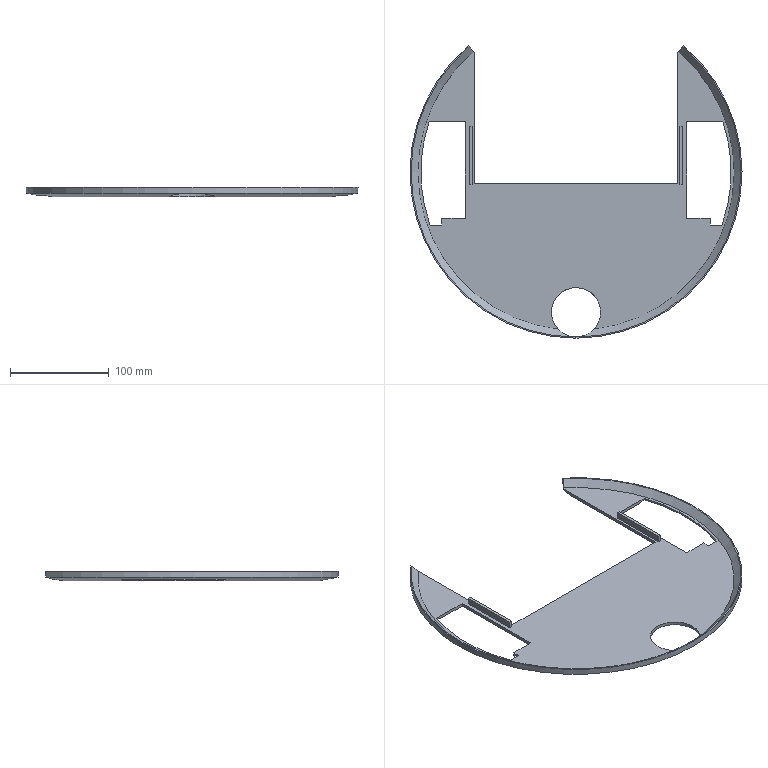Component | NX | BOTTOM_SHELL | 1 solid | 34 faces | volume 142559 mm3 | plane 28 | cylinder 4 | cone 2 | commonest cylinder face diameters 314.52 x2 336.354 x1 50 x1